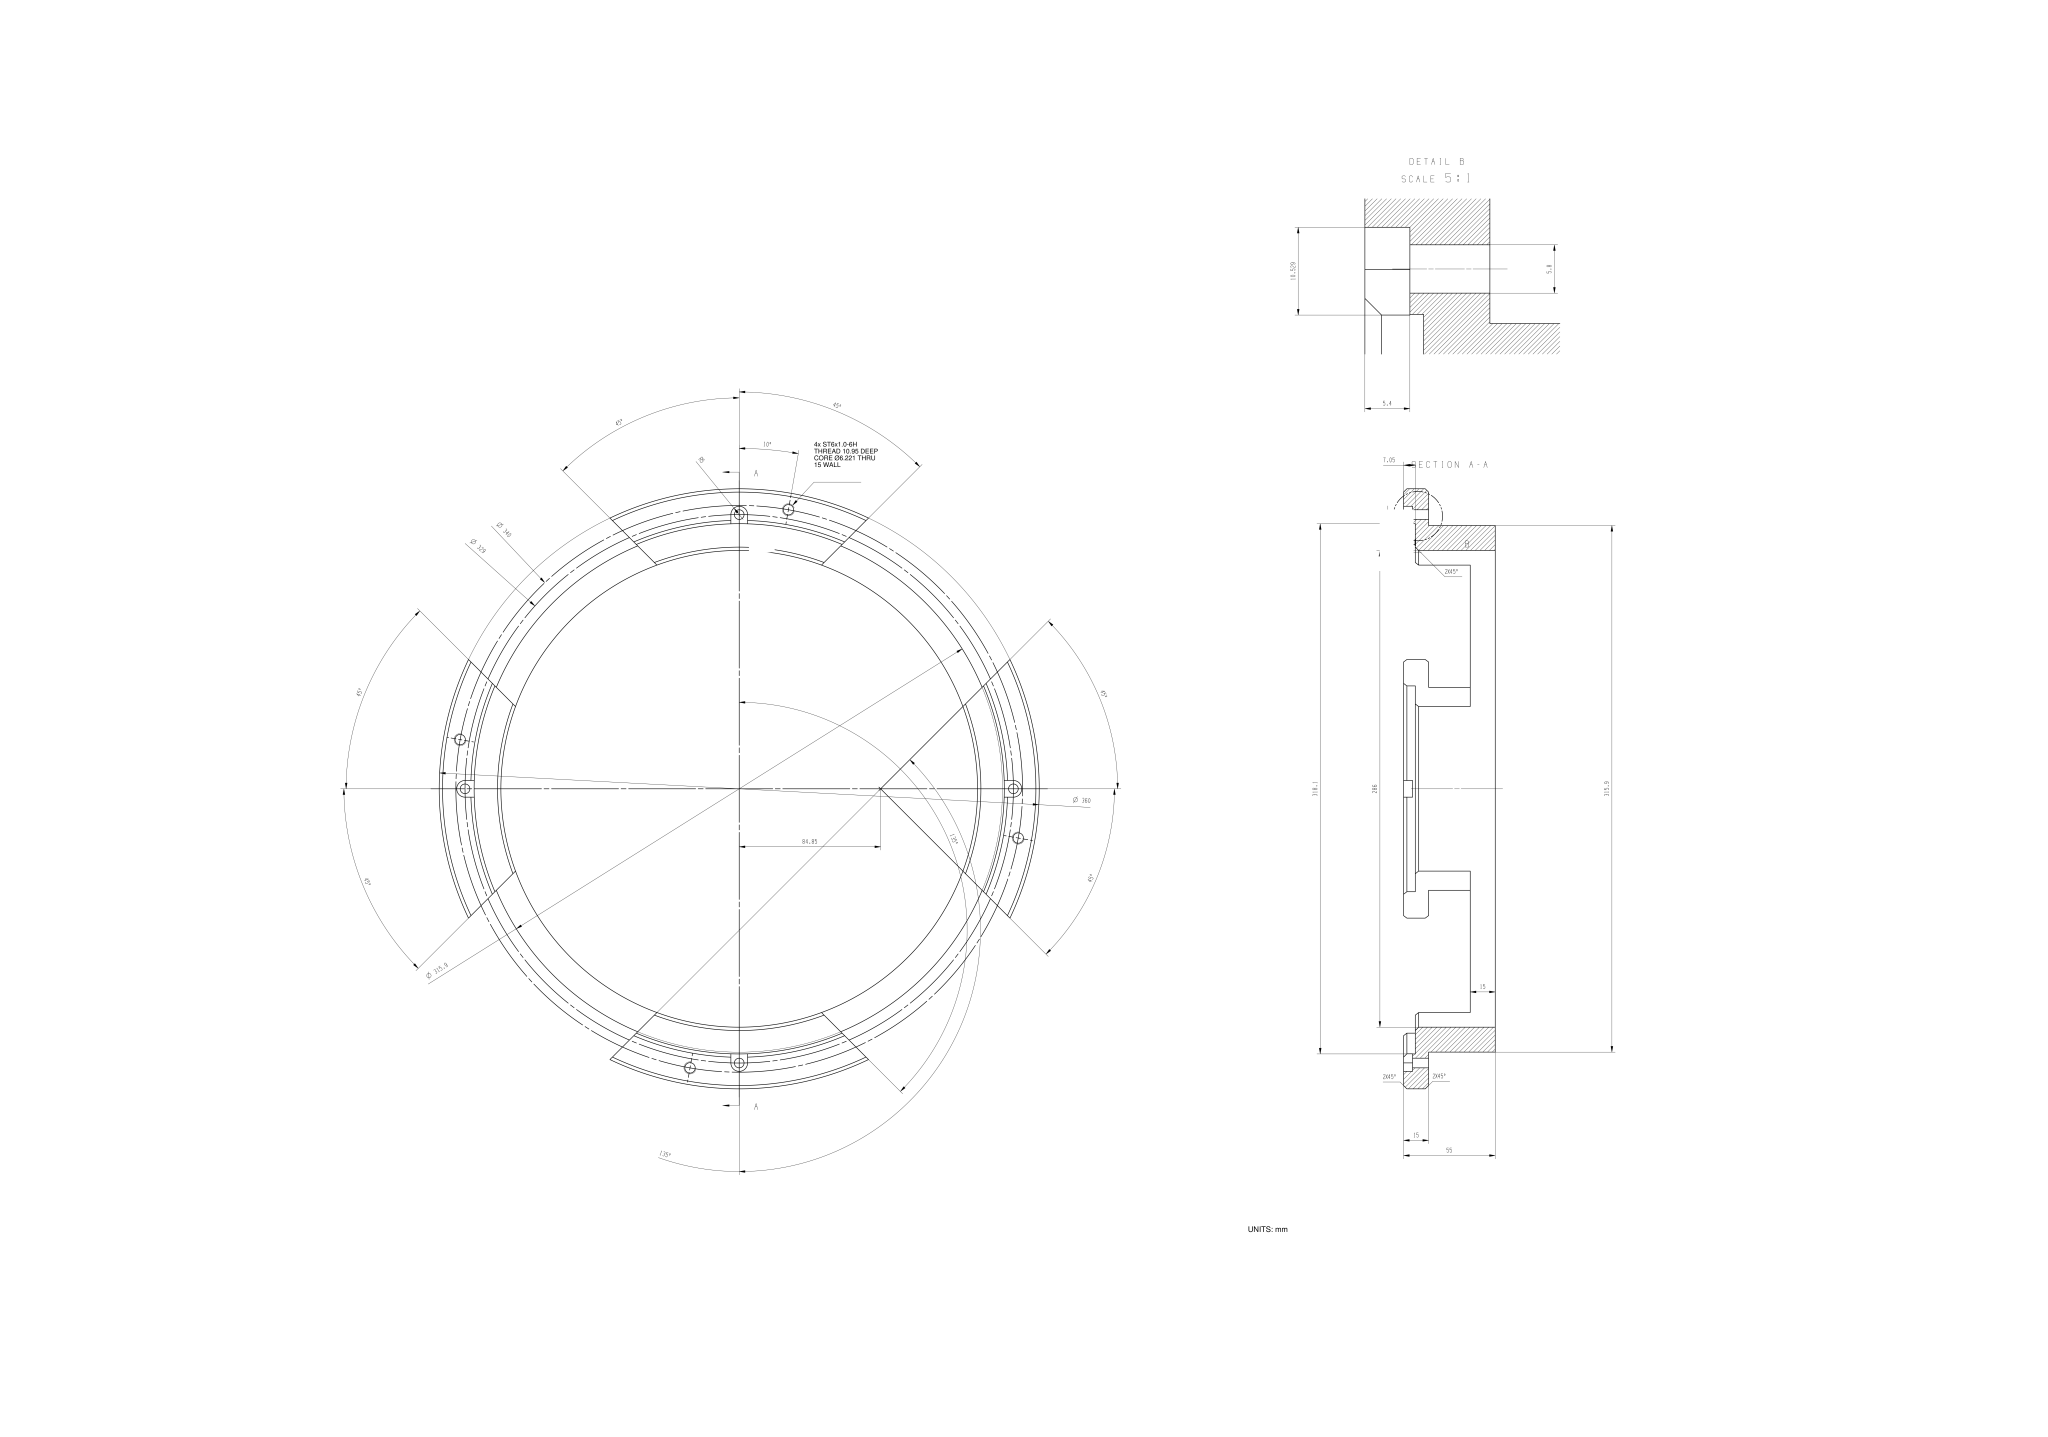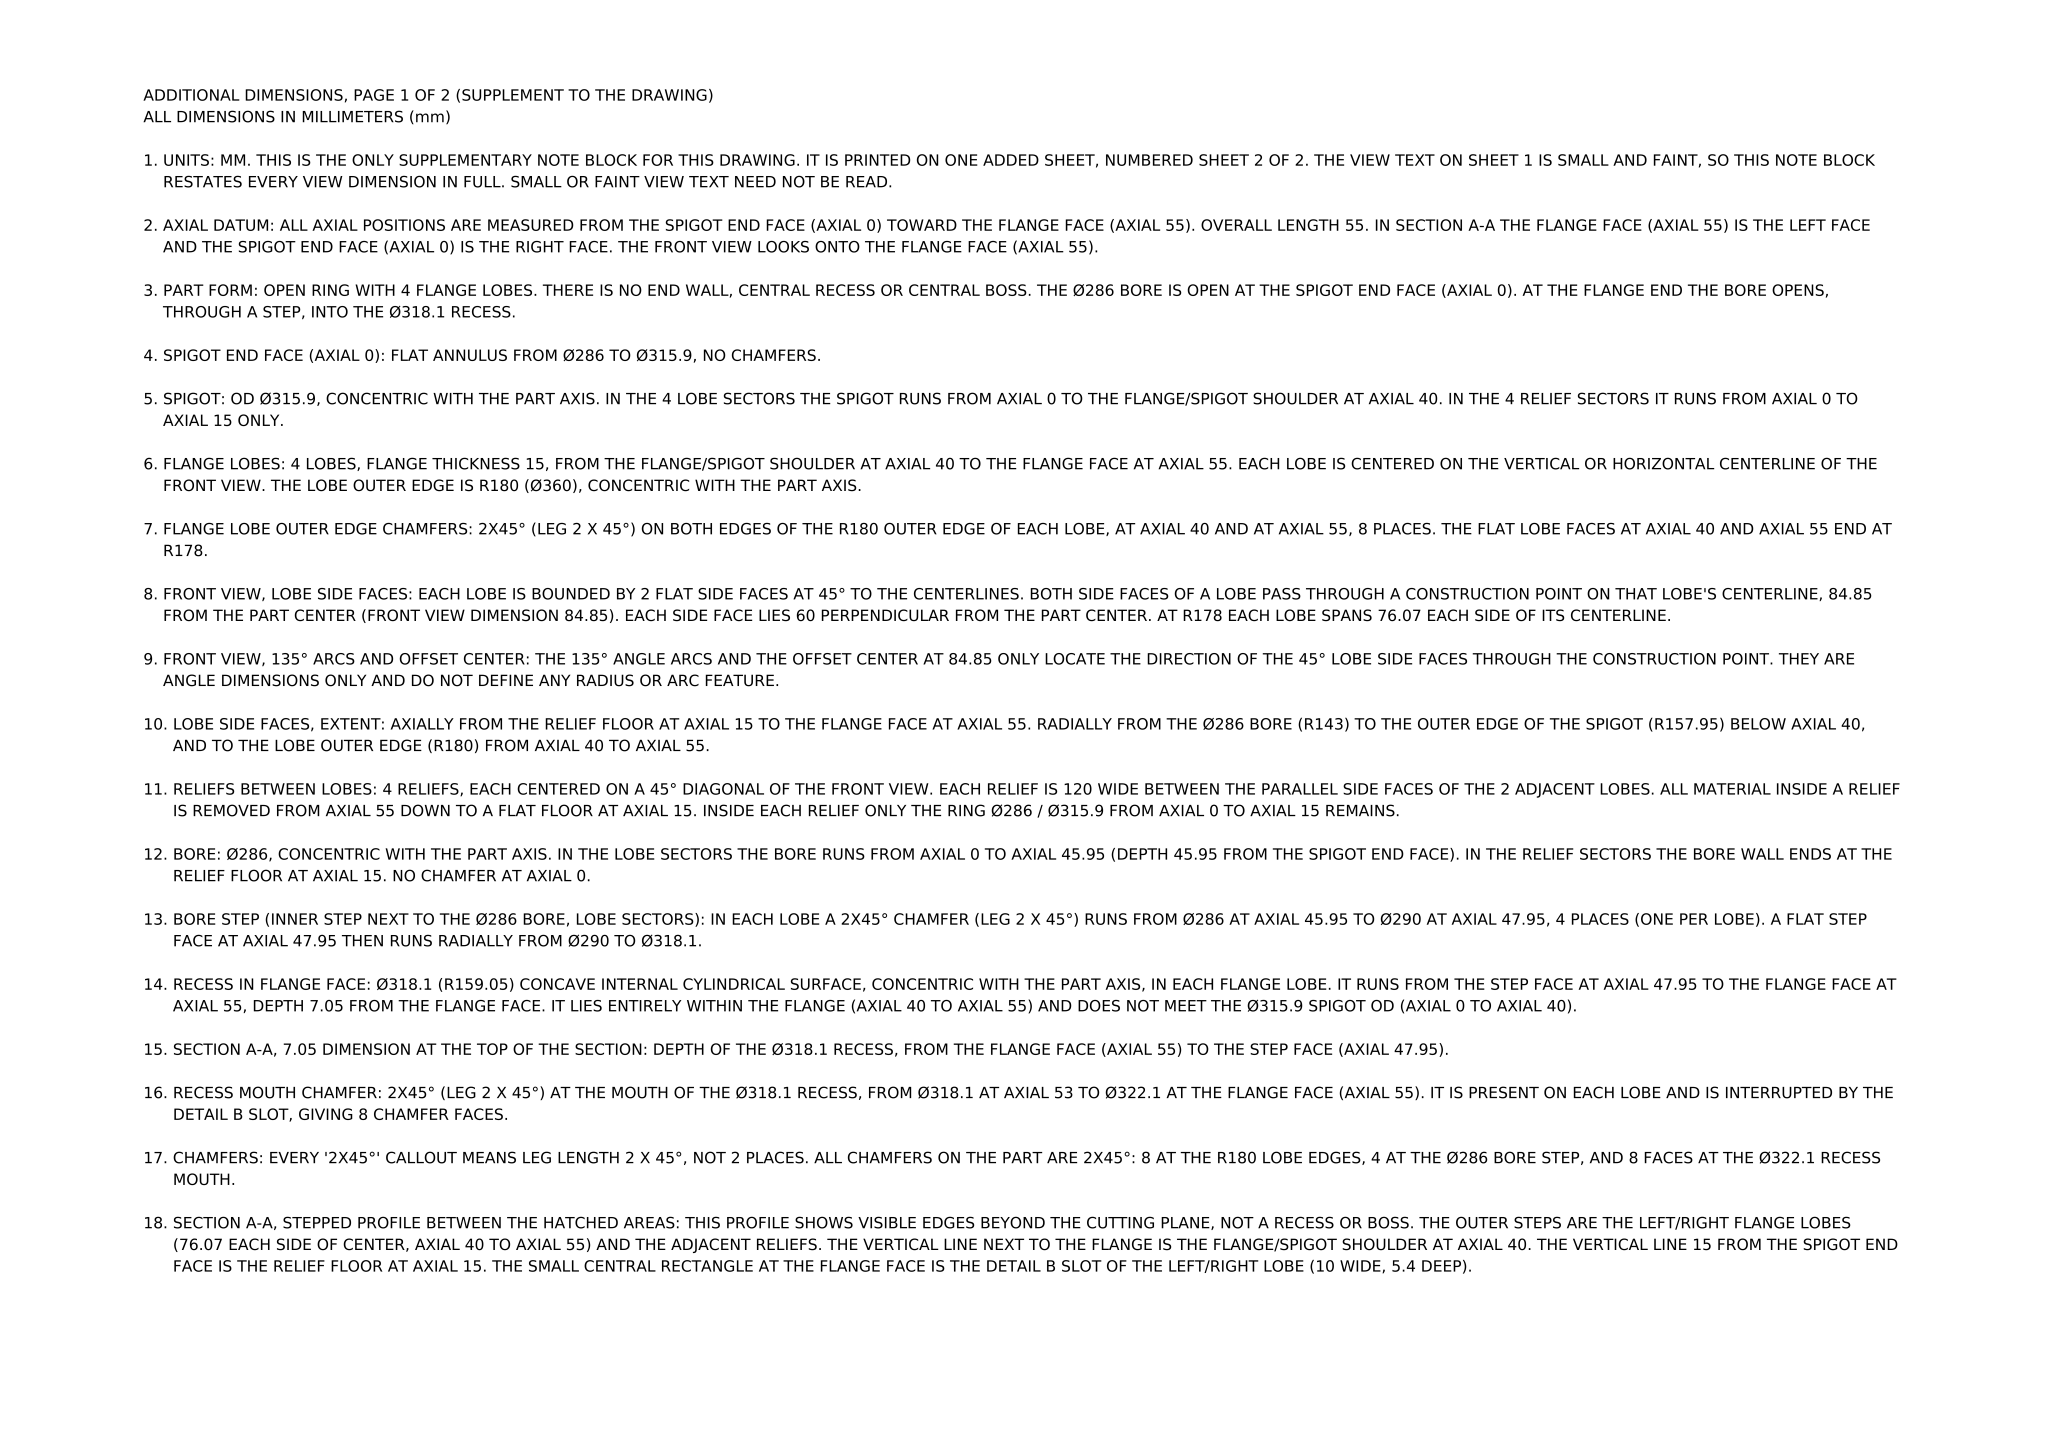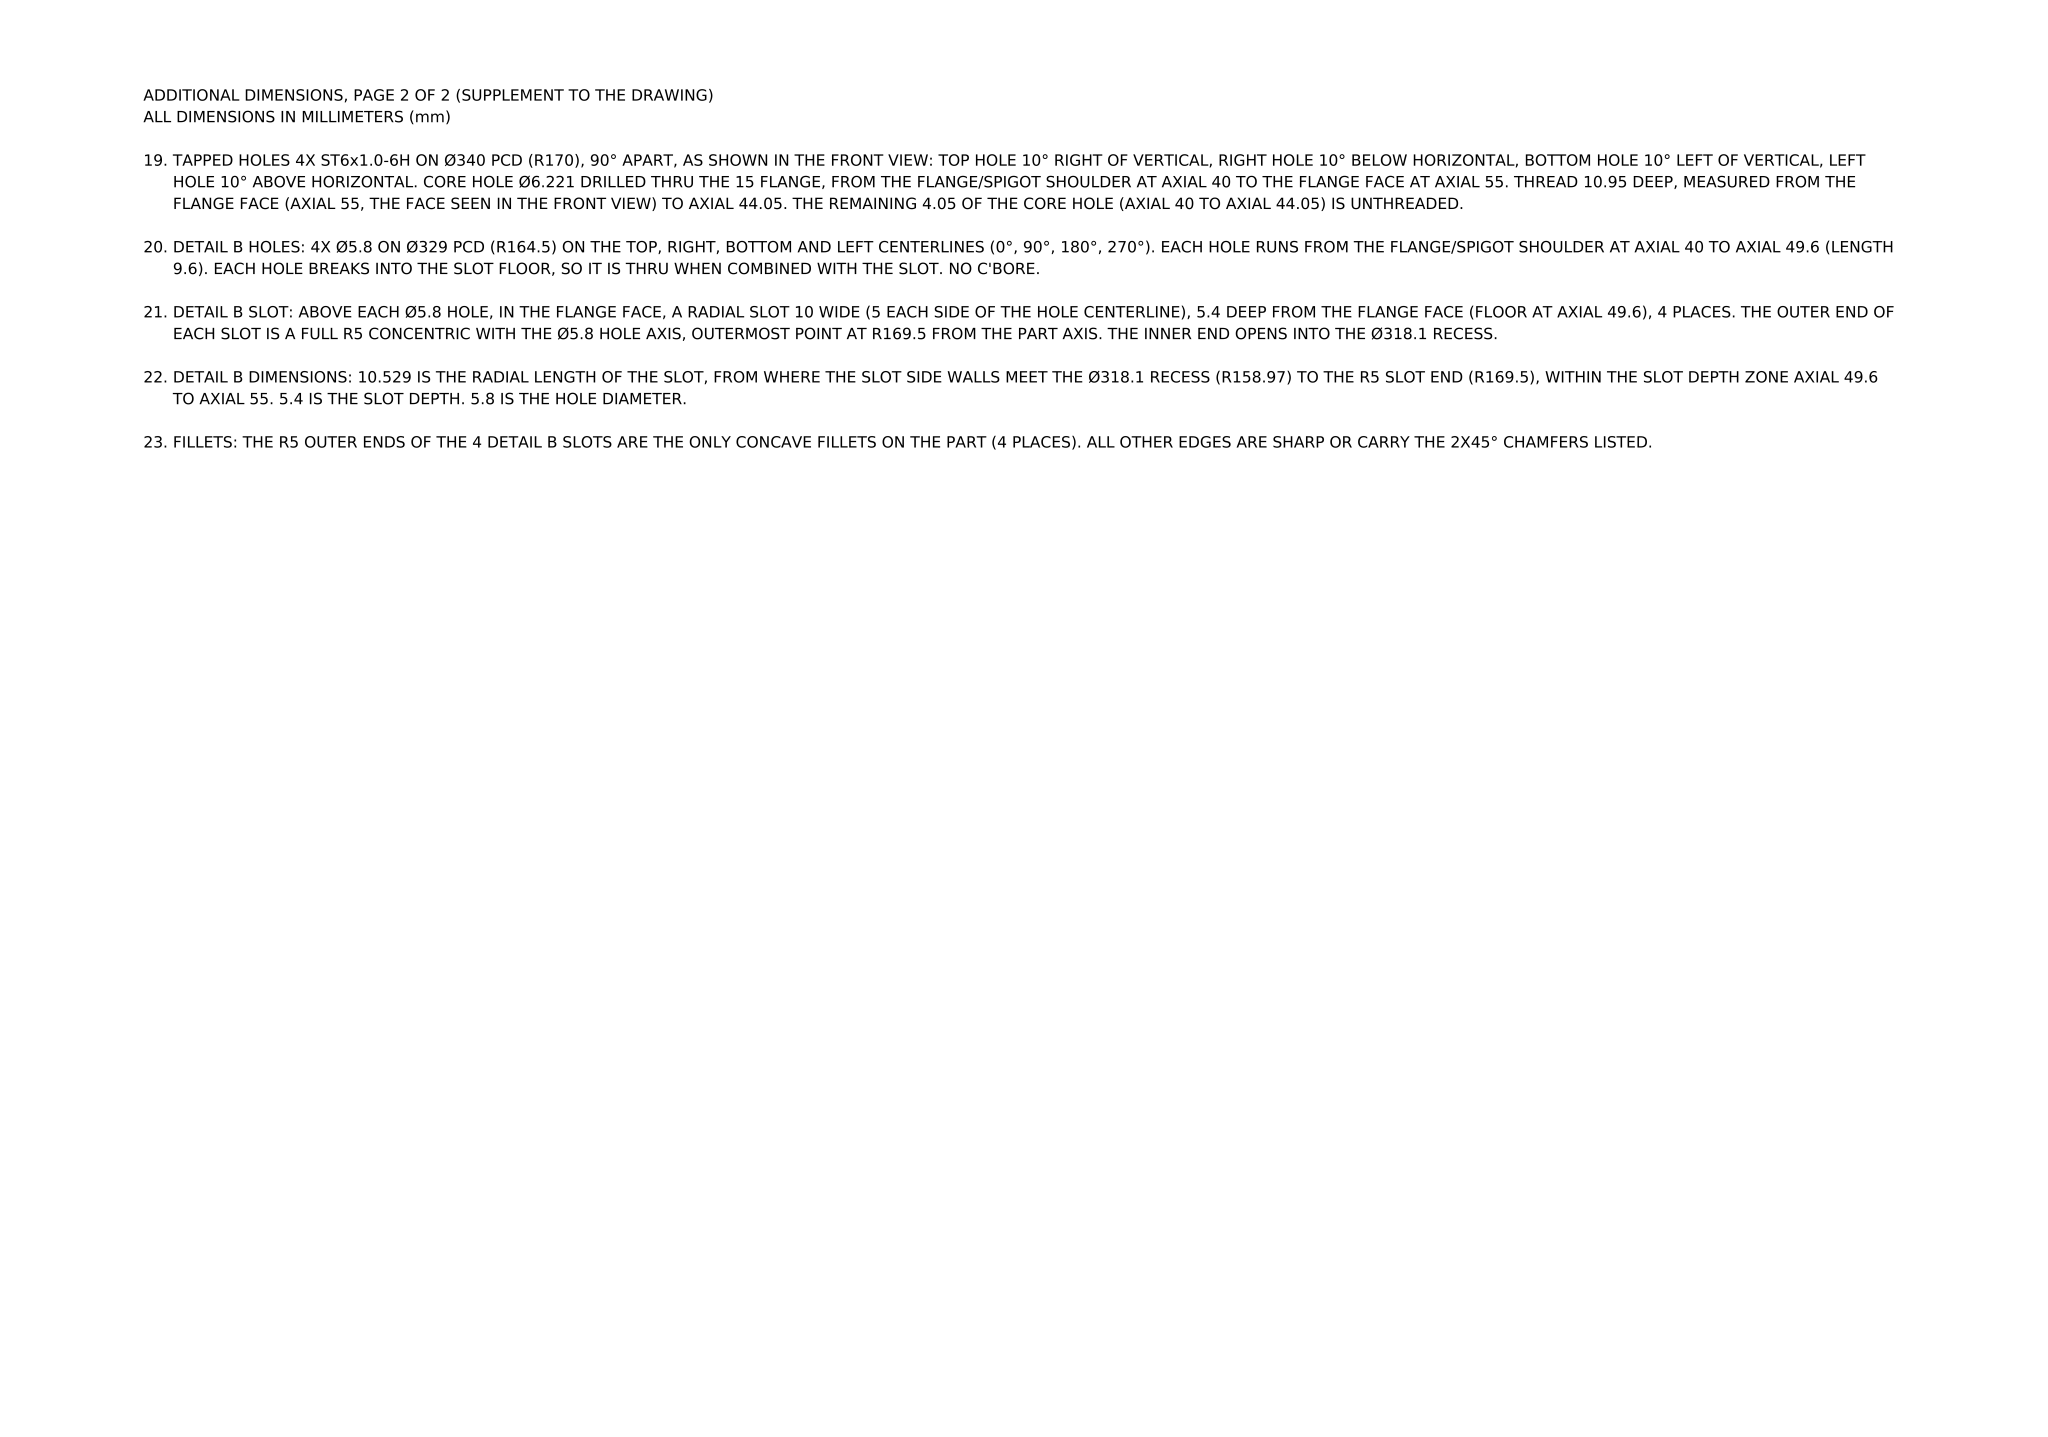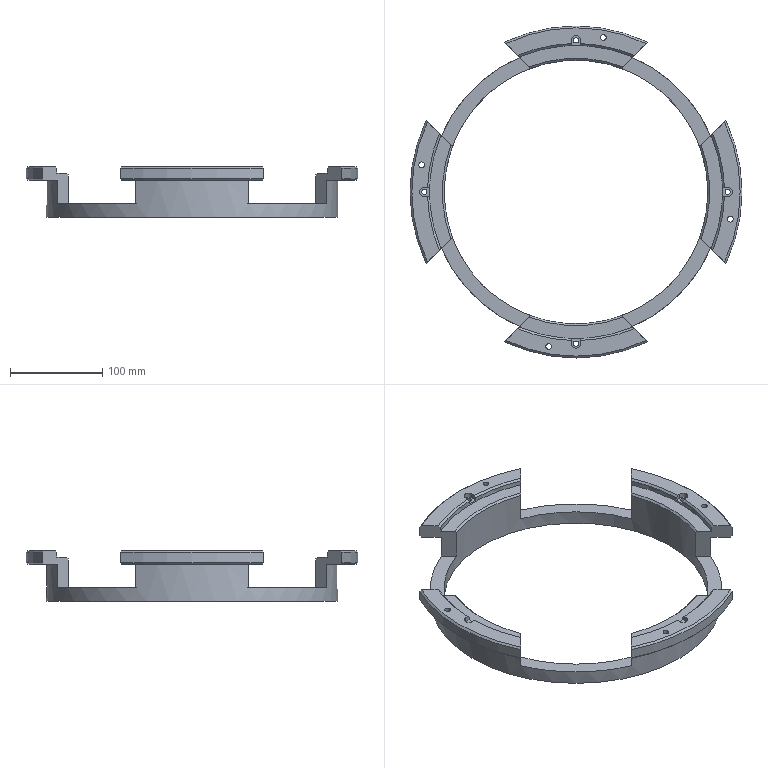Part | NX | mm | 1 solid | 79 faces | box 360 x 360 x 55 mm | volume 610298 mm3 | plane 37 | cylinder 22 | cone 20 | commonest cylinder face diameters 360 x4 318.1 x4 6.221 x4 5.8 x4 10 x4 315.9 x1 286 x1